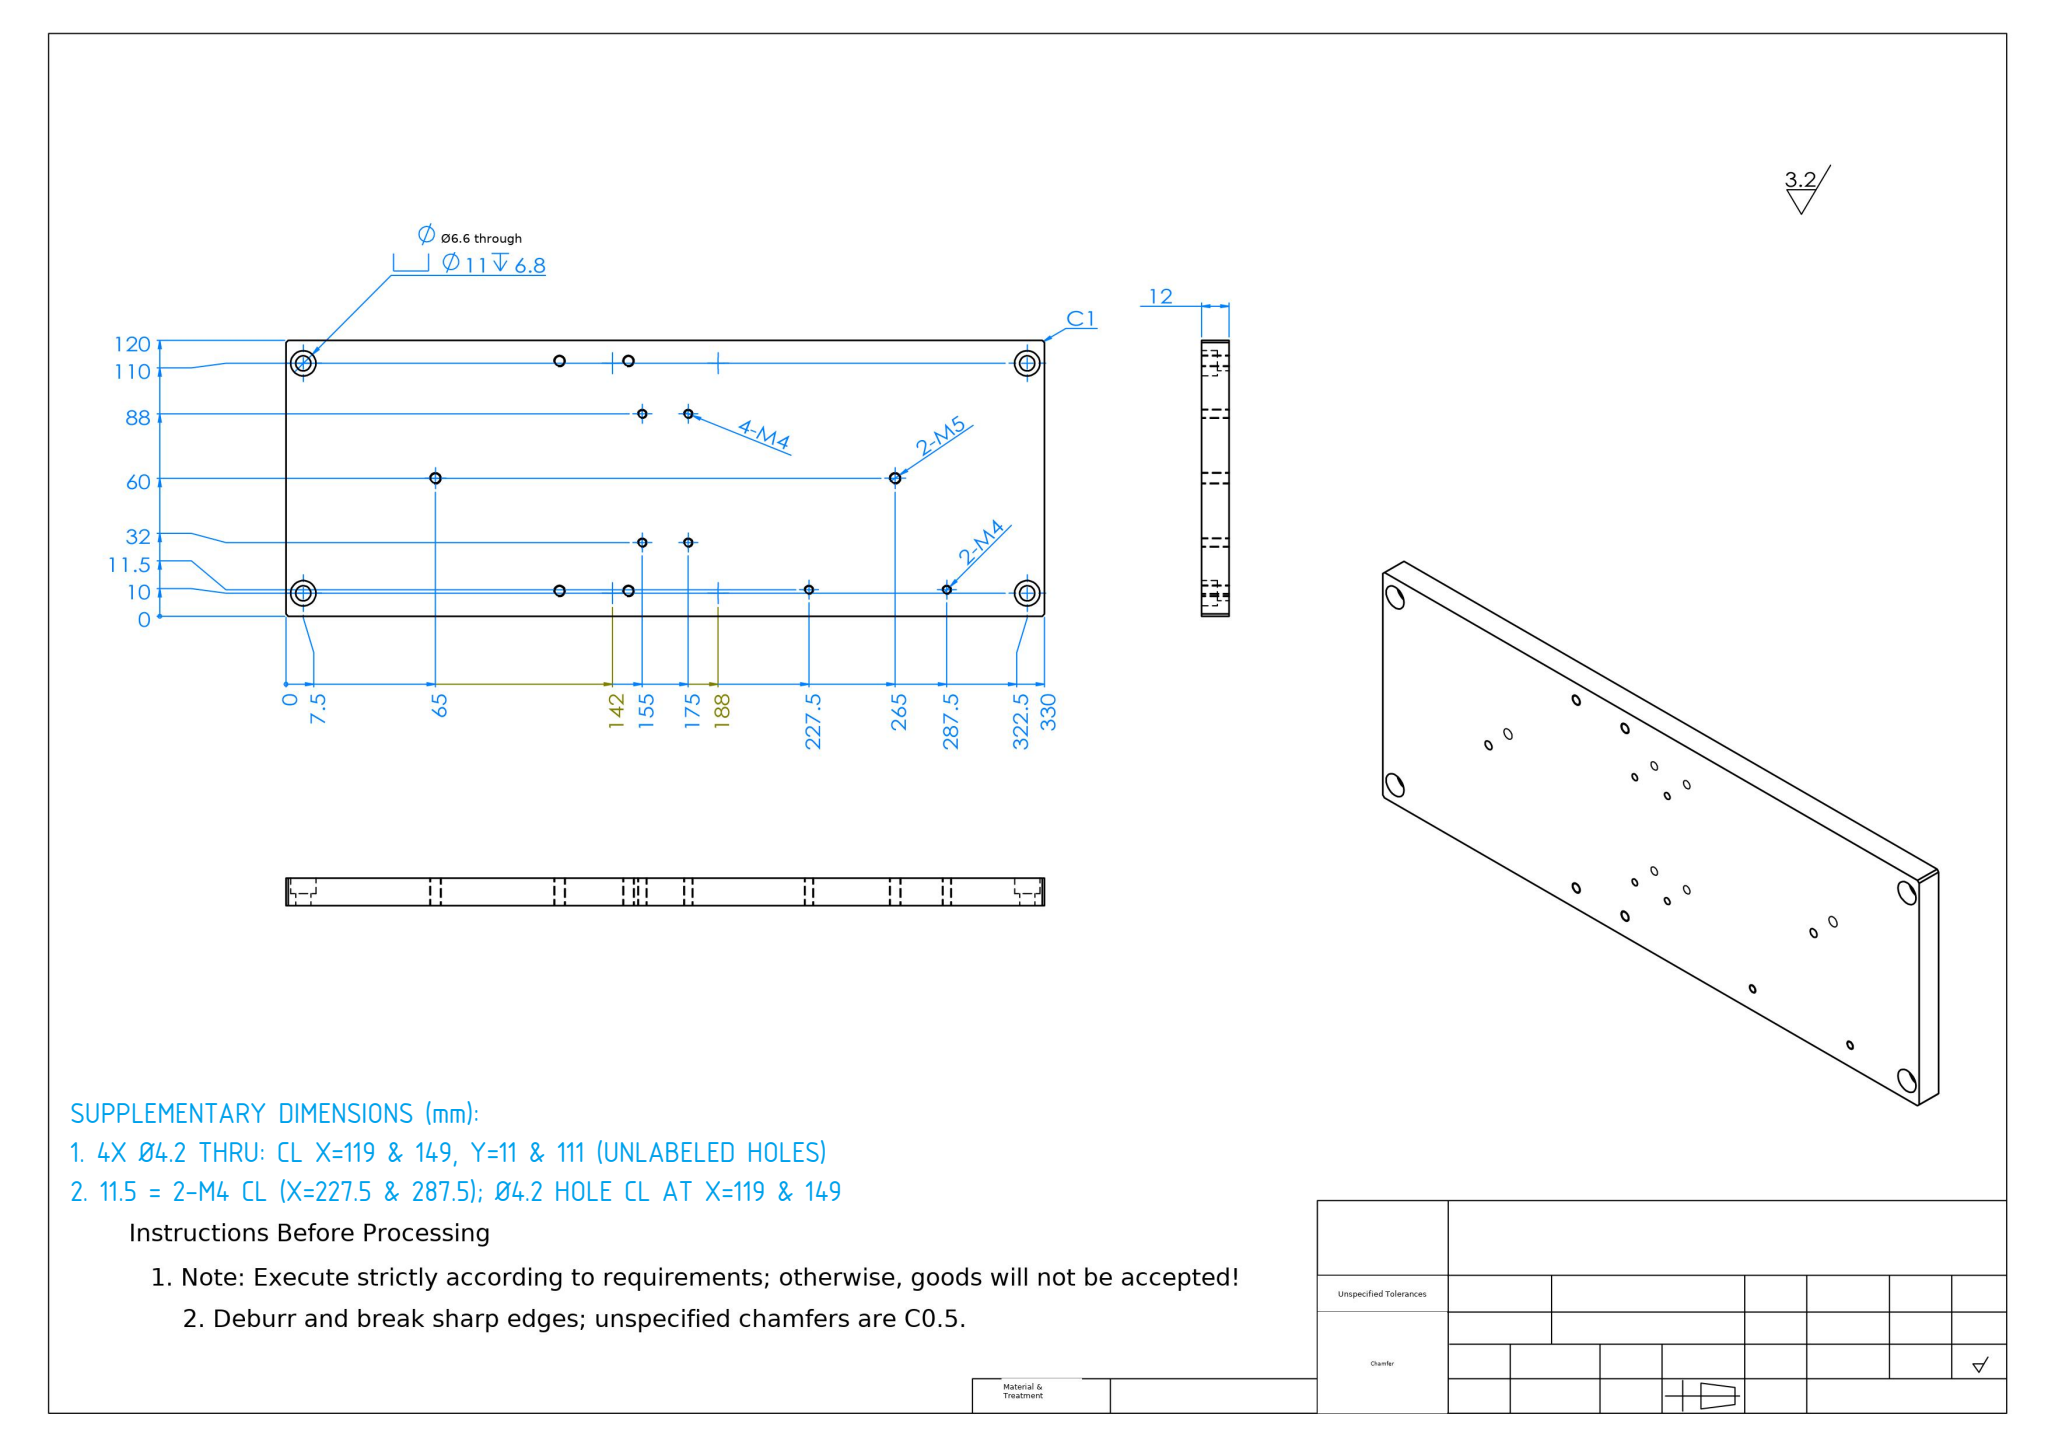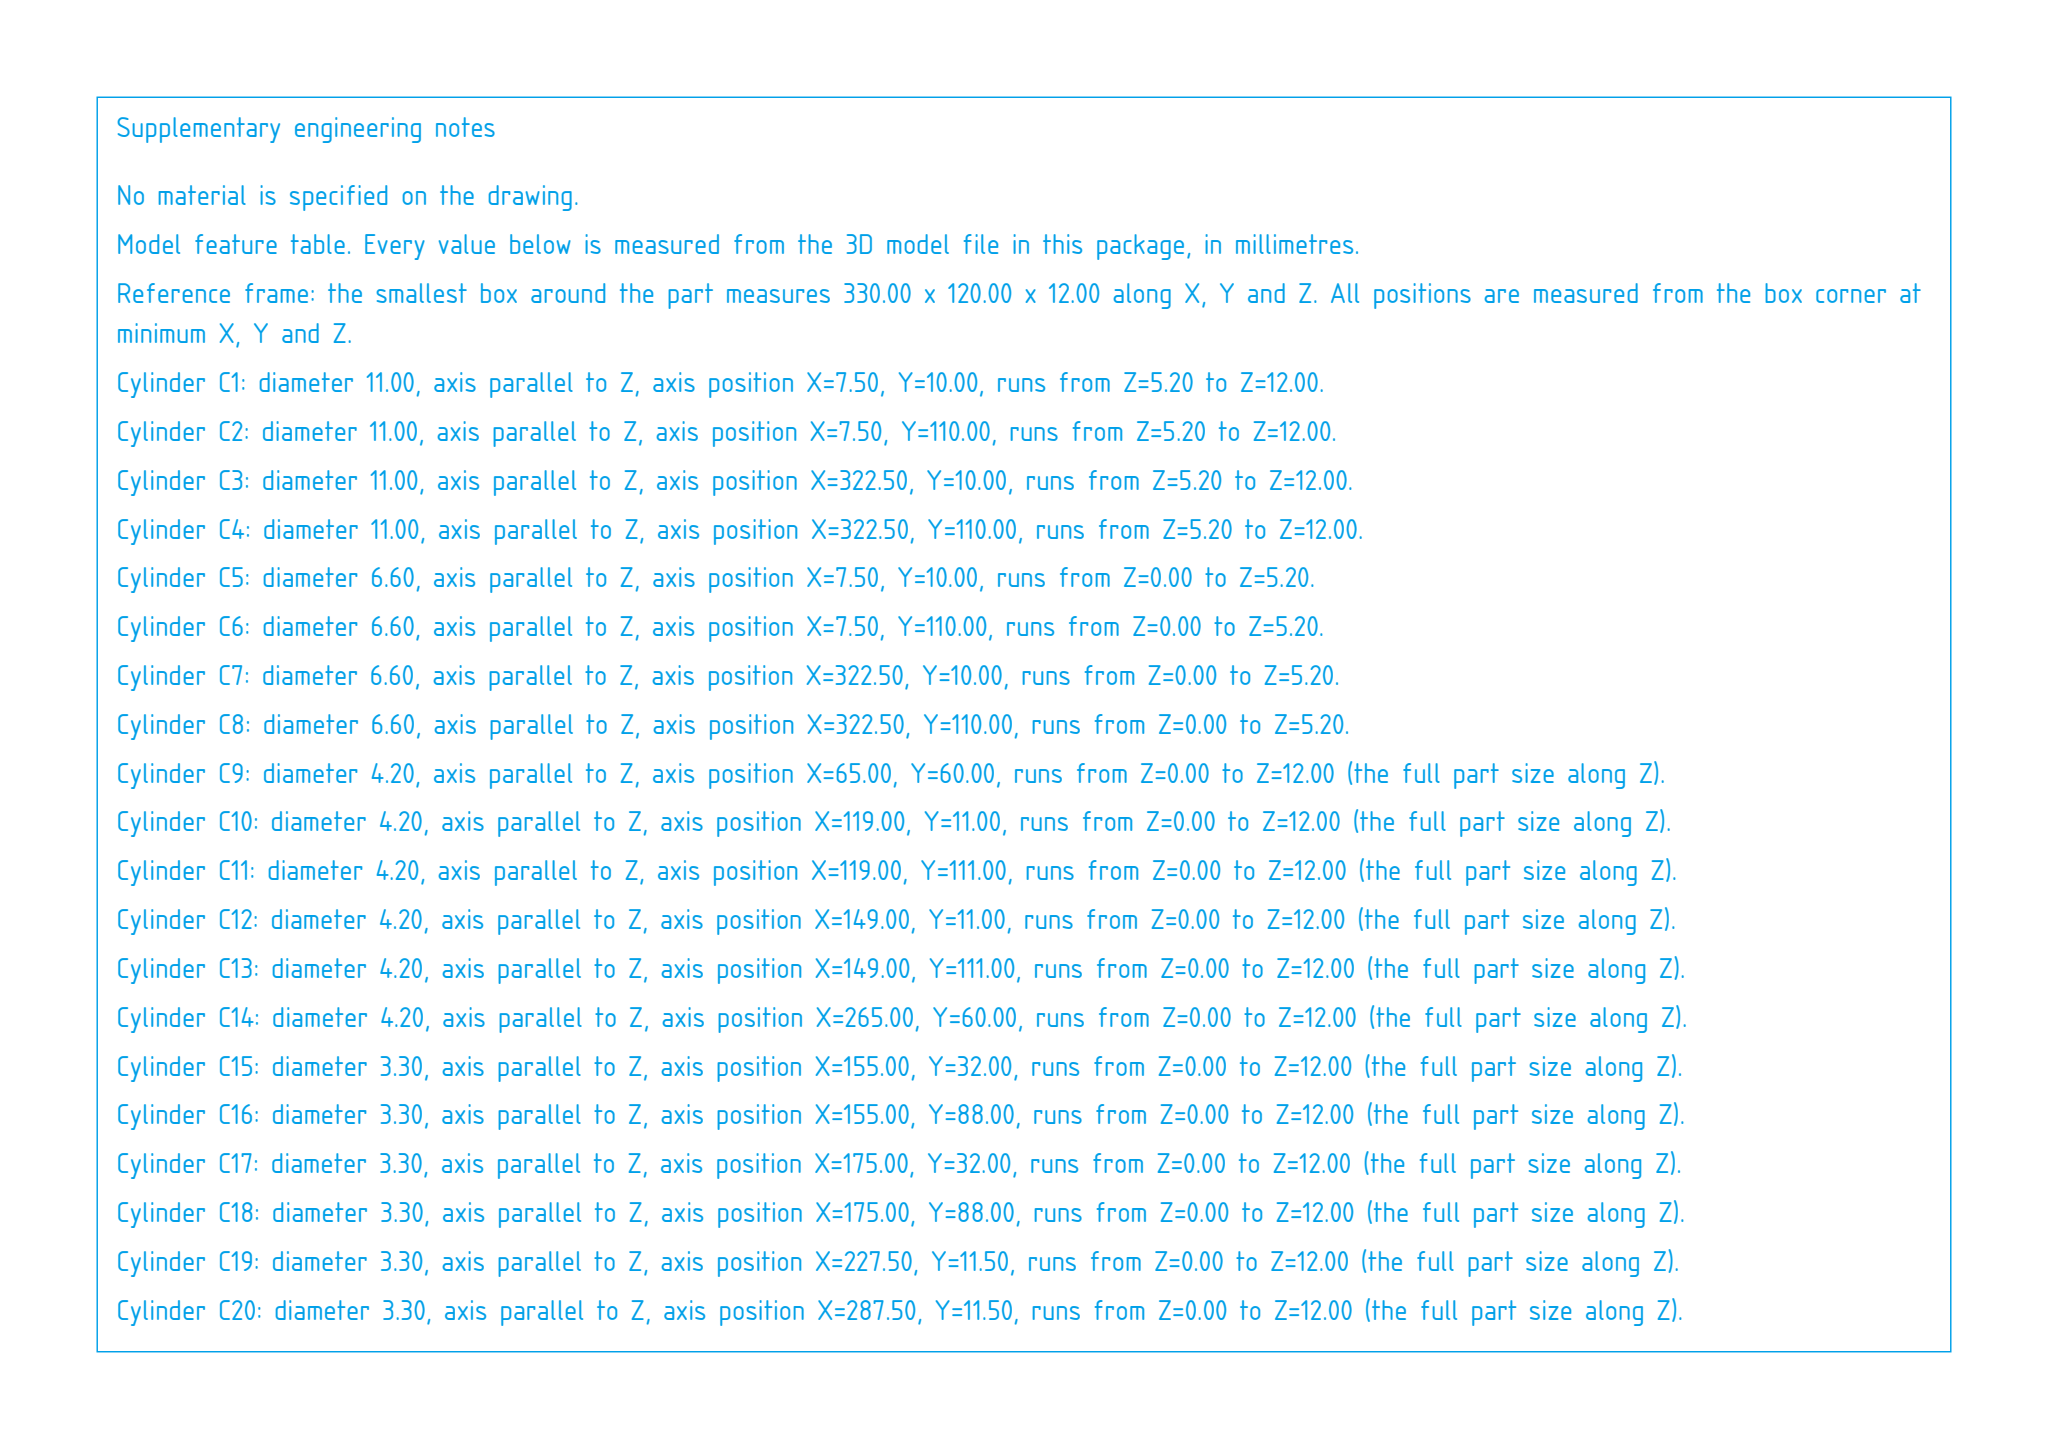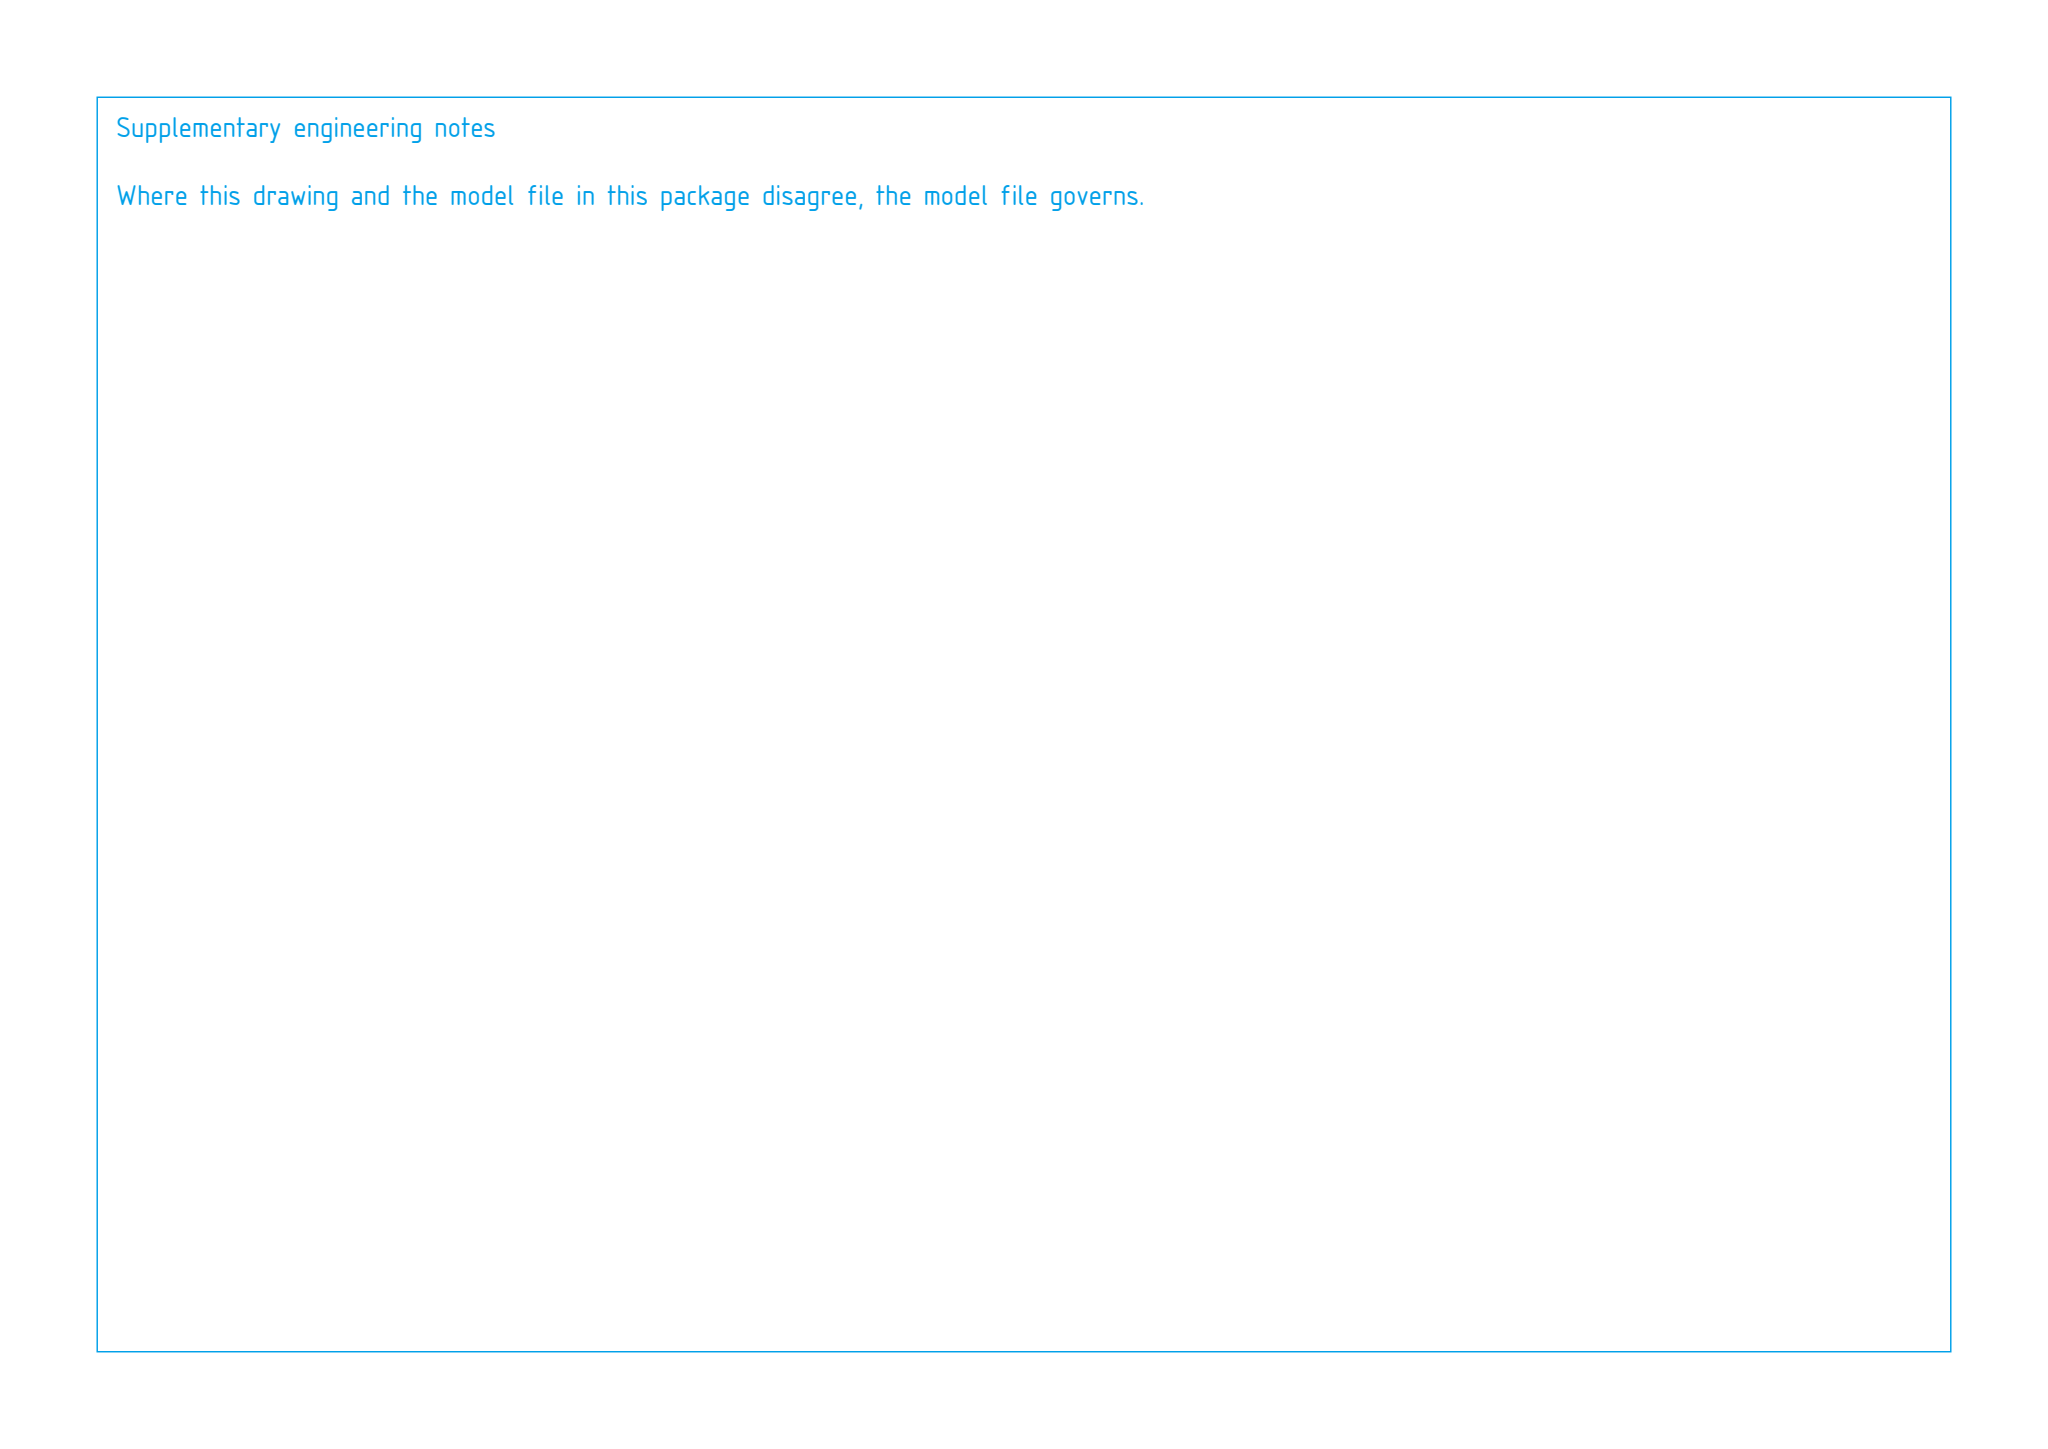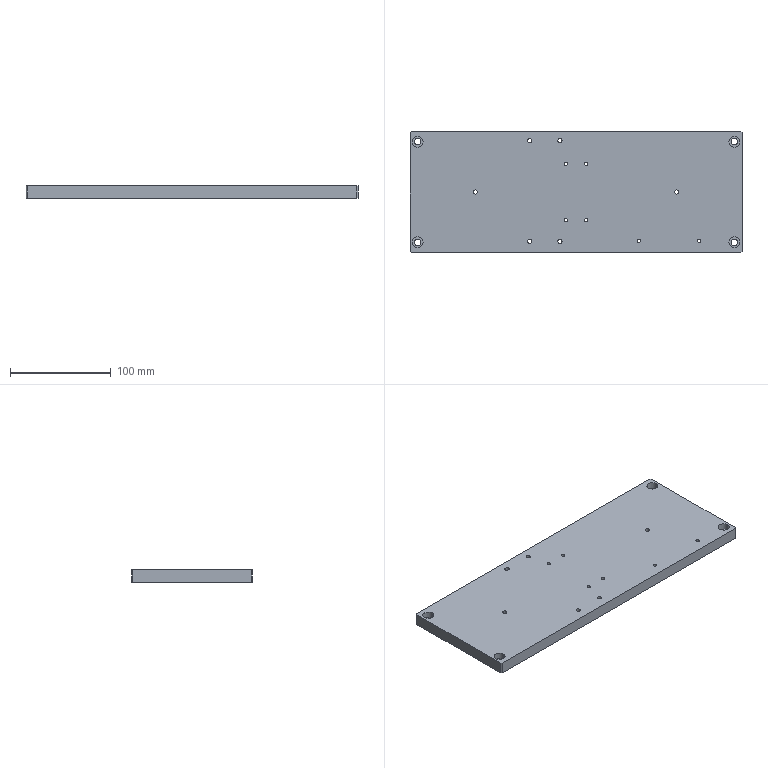Part | SolidWorks | mm | 1 solid | 54 faces | box 330 x 120 x 12 mm | volume 470266 mm3 | cylinder 40 | plane 14 | commonest cylinder face diameters 4.2 x12 3.3 x12 11 x8 6.6 x8
build123d program:
from build123d import *

# Parameters (mm, degrees)
SKETCH1_W                                         = 330
SKETCH1_H                                         = 120
BOSS_EXTRUDE1_DEPTH                               = 6
CHAMFER1_SIZE                                     = 1
HOLE_SIZE_ACCORDING_TO_HEXAGON_SOCKET_D           = 6.6
HOLE_SIZE_ACCORDING_TO_HEXAGON_SOCKET_CBORE_D     = 11
HOLE_SIZE_ACCORDING_TO_HEXAGON_SOCKET_CBORE_DEPTH = 6.8
M4_TAPPED_HOLE1_D                                 = 3.3
M5_TAPPED_HOLE1_D                                 = 4.2
M4_TAPPED_HOLE2_D                                 = 3.3
M5_TAPPED_HOLE3_D                                 = 4.2


with BuildPart() as part:
    # Sketch1 → Boss-Extrude1 (new, symmetric)
    with BuildSketch(Plane.XY):
        Rectangle(SKETCH1_W, SKETCH1_H)
    extrude(amount=BOSS_EXTRUDE1_DEPTH, both=True)

    # Chamfer1
    chamfer1_edges = [part.edges().sort_by_distance(p)[0] for p in [
        (165, -60, 0),
        (-165, -60, 0),
        (-165, 60, 0),
        (165, 60, 0),
    ]]
    chamfer(chamfer1_edges, length=CHAMFER1_SIZE)

    # Hole Size _ according to_ Hexagon Socket (through all)
    with Locations(Plane.XY.offset(6)):
        with Locations((-157.5, 50), (-157.5, -50), (157.5, -50), (157.5, 50)):
            CounterBoreHole(HOLE_SIZE_ACCORDING_TO_HEXAGON_SOCKET_D / 2, HOLE_SIZE_ACCORDING_TO_HEXAGON_SOCKET_CBORE_D / 2, HOLE_SIZE_ACCORDING_TO_HEXAGON_SOCKET_CBORE_DEPTH)

    # M4 Tapped Hole1 (through all)
    with Locations(Plane(origin=(0, 0, -6), x_dir=(-1, 0, 0), z_dir=(0, 0, -1))):
        with Locations((-10, 28), (10, 28), (-10, -28), (10, -28)):
            Hole(M4_TAPPED_HOLE1_D / 2)

    # M5 Tapped Hole1 (through all)
    with Locations(Plane(origin=(0, 0, -6), x_dir=(-1, 0, 0), z_dir=(0, 0, -1))):
        with Locations((-100, 0), (100, 0)):
            Hole(M5_TAPPED_HOLE1_D / 2)

    # M4 Tapped Hole2 (through all)
    with Locations(Plane.XY.offset(6)):
        with Locations((62.5, -48.5), (122.5, -48.5)):
            Hole(M4_TAPPED_HOLE2_D / 2)

    # M5 Tapped Hole3 (through all)
    with Locations(Plane.XY.offset(6)):
        with Locations((-16, 51), (-46, 51), (-46, -49), (-16, -49)):
            Hole(M5_TAPPED_HOLE3_D / 2)


solid = part.part